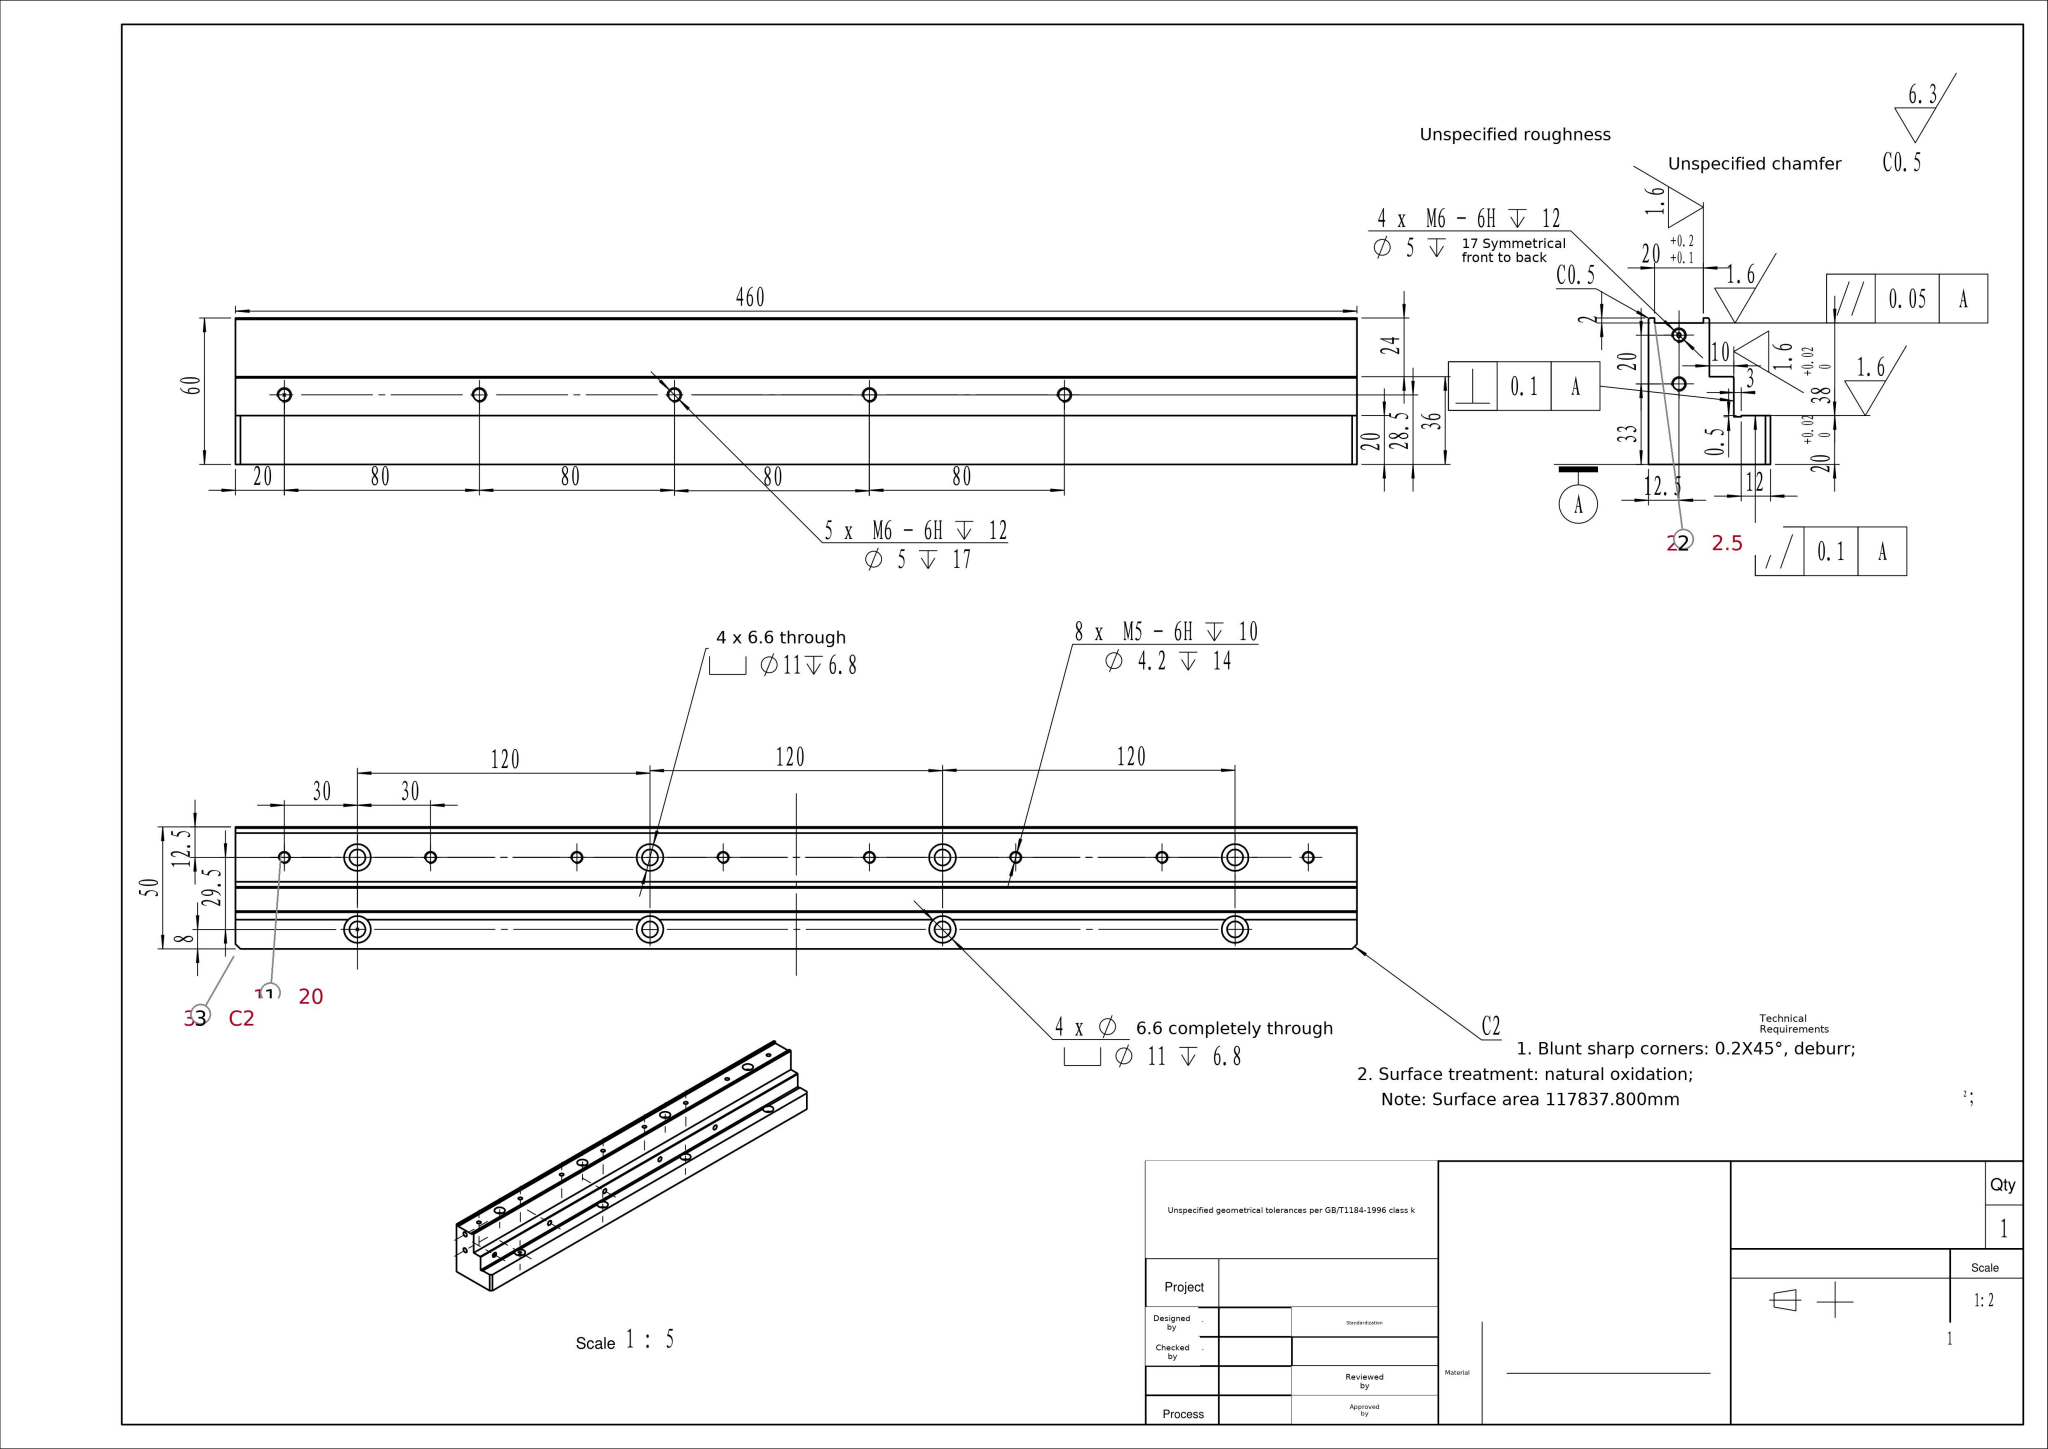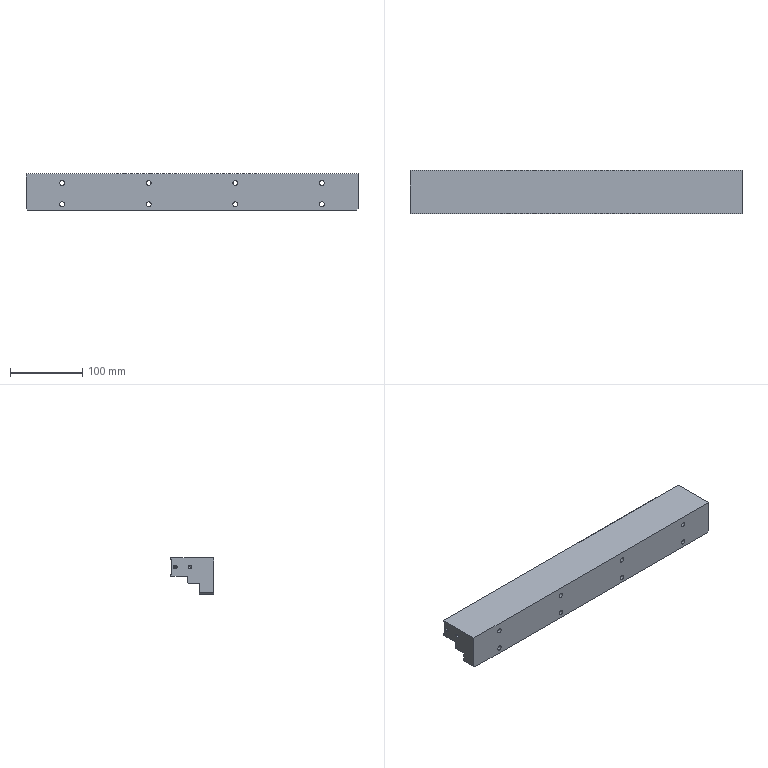Part | SolidWorks | mm | 1 solid | 133 faces | box 460 x 60 x 50 mm | volume 955600 mm3 | cylinder 66 | cone 34 | plane 33 | commonest cylinder face diameters 5 x18 6.6 x16 11 x16 4.2 x16